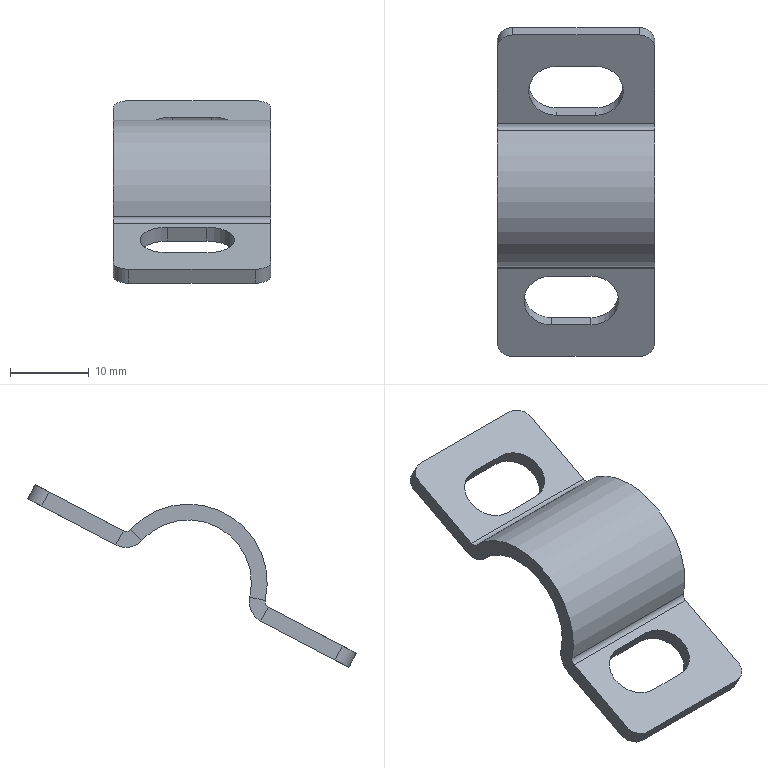Component | SolidWorks | SpringSnap-1 | 1 solid | 34 faces | box 20 x 41.66 x 23.15 mm | volume 1836 mm3 | plane 20 | cylinder 14 | commonest cylinder face diameters 7 x4 4 x4 5.473 x2 1.473 x2 16 x1 20 x1
STEP:
#1=COLOUR_RGB('',0.7922,0.8196,0.9333);
#2=FILL_AREA_STYLE_COLOUR('',#1);
#3=FILL_AREA_STYLE('',(#2));
#4=SURFACE_STYLE_FILL_AREA(#3);
#5=SURFACE_SIDE_STYLE('',(#4));
#6=SURFACE_STYLE_USAGE(.BOTH.,#5);
#7=PRESENTATION_STYLE_ASSIGNMENT((#6));
#8=CARTESIAN_POINT('',(-8.595,-0.65,7.005));
#9=VERTEX_POINT('',#8);
#10=CARTESIAN_POINT('',(-8.595,-0.592,7.058));
#11=VERTEX_POINT('',#10);
#12=CARTESIAN_POINT('',(-8.595,-0.65,7.005));
#13=DIRECTION('',(-0.,0.7377,0.6751));
#14=VECTOR('',#13,39.37);
#15=LINE('',#12,#14);
#16=EDGE_CURVE('',#9,#11,#15,.T.);
#17=ORIENTED_EDGE('',*,*,#16,.F.);
#18=CARTESIAN_POINT('',(-8.595,-0.5205,6.982));
#19=VERTEX_POINT('',#18);
#20=CARTESIAN_POINT('',(-8.595,-0.5706,7.078));
#21=DIRECTION('',(-1.,-0.,-0.));
#22=DIRECTION('',(0.,-0.8854,-0.4648));
#23=AXIS2_PLACEMENT_3D('',#20,#21,#22);
#24=CIRCLE('',#23,0.1077);
#25=EDGE_CURVE('',#19,#9,#24,.T.);
#26=ORIENTED_EDGE('',*,*,#25,.F.);
#27=CARTESIAN_POINT('',(-8.595,-0.5571,7.052));
#28=VERTEX_POINT('',#27);
#29=CARTESIAN_POINT('',(-8.595,-0.5571,7.052));
#30=DIRECTION('',(-0.,0.4648,-0.8854));
#31=VECTOR('',#30,39.37);
#32=LINE('',#29,#31);
#33=EDGE_CURVE('',#28,#19,#32,.T.);
#34=ORIENTED_EDGE('',*,*,#33,.F.);
#35=CARTESIAN_POINT('',(-8.595,-0.5706,7.078));
#36=DIRECTION('',(-1.,-0.,-0.));
#37=DIRECTION('',(0.,-0.8854,-0.4648));
#38=AXIS2_PLACEMENT_3D('',#35,#36,#37);
#39=CIRCLE('',#38,0.029);
#40=EDGE_CURVE('',#28,#11,#39,.T.);
#41=ORIENTED_EDGE('',*,*,#40,.T.);
#42=EDGE_LOOP('',(#17,#26,#34,#41));
#43=FACE_OUTER_BOUND('',#42,.T.);
#44=CARTESIAN_POINT('',(-8.595,-0.65,7.005));
#45=DIRECTION('',(1.,0.,0.));
#46=DIRECTION('',(0.,-0.8854,-0.4648));
#47=AXIS2_PLACEMENT_3D('',#44,#45,#46);
#48=PLANE('',#47);
#49=ADVANCED_FACE('',(#43),#48,.T.);
#50=CARTESIAN_POINT('',(-8.595,-1.189,6.722));
#51=VERTEX_POINT('',#50);
#52=CARTESIAN_POINT('',(-8.595,-0.8824,6.792));
#53=DIRECTION('',(1.,0.,0.));
#54=DIRECTION('',(0.,-0.8854,-0.4648));
#55=AXIS2_PLACEMENT_3D('',#52,#53,#54);
#56=CIRCLE('',#55,0.315);
#57=EDGE_CURVE('',#9,#51,#56,.T.);
#58=ORIENTED_EDGE('',*,*,#57,.F.);
#59=ORIENTED_EDGE('',*,*,#16,.T.);
#60=CARTESIAN_POINT('',(-8.595,-1.266,6.704));
#61=VERTEX_POINT('',#60);
#62=CARTESIAN_POINT('',(-8.595,-0.8824,6.792));
#63=DIRECTION('',(1.,0.,0.));
#64=DIRECTION('',(0.,-0.8854,-0.4648));
#65=AXIS2_PLACEMENT_3D('',#62,#63,#64);
#66=CIRCLE('',#65,0.3937);
#67=EDGE_CURVE('',#11,#61,#66,.T.);
#68=ORIENTED_EDGE('',*,*,#67,.T.);
#69=CARTESIAN_POINT('',(-8.595,-1.266,6.704));
#70=DIRECTION('',(-0.,0.9746,0.2238));
#71=VECTOR('',#70,39.37);
#72=LINE('',#69,#71);
#73=EDGE_CURVE('',#61,#51,#72,.T.);
#74=ORIENTED_EDGE('',*,*,#73,.T.);
#75=EDGE_LOOP('',(#58,#59,#68,#74));
#76=FACE_OUTER_BOUND('',#75,.T.);
#77=CARTESIAN_POINT('',(-8.595,-0.5571,7.052));
#78=DIRECTION('',(1.,0.,0.));
#79=DIRECTION('',(0.,-0.8854,-0.4648));
#80=AXIS2_PLACEMENT_3D('',#77,#78,#79);
#81=PLANE('',#80);
#82=ADVANCED_FACE('',(#76),#81,.T.);
#83=CARTESIAN_POINT('',(-9.383,-0.5205,6.982));
#84=VERTEX_POINT('',#83);
#85=CARTESIAN_POINT('',(-9.383,-0.5571,7.052));
#86=VERTEX_POINT('',#85);
#87=CARTESIAN_POINT('',(-9.383,-0.5205,6.982));
#88=DIRECTION('',(0.,-0.4648,0.8854));
#89=VECTOR('',#88,39.37);
#90=LINE('',#87,#89);
#91=EDGE_CURVE('',#84,#86,#90,.T.);
#92=ORIENTED_EDGE('',*,*,#91,.F.);
#93=CARTESIAN_POINT('',(-9.383,-0.65,7.005));
#94=VERTEX_POINT('',#93);
#95=CARTESIAN_POINT('',(-9.383,-0.5706,7.078));
#96=DIRECTION('',(-1.,-0.,-0.));
#97=DIRECTION('',(0.,-0.8854,-0.4648));
#98=AXIS2_PLACEMENT_3D('',#95,#96,#97);
#99=CIRCLE('',#98,0.1077);
#100=EDGE_CURVE('',#84,#94,#99,.T.);
#101=ORIENTED_EDGE('',*,*,#100,.T.);
#102=CARTESIAN_POINT('',(-9.383,-0.592,7.058));
#103=VERTEX_POINT('',#102);
#104=CARTESIAN_POINT('',(-9.383,-0.592,7.058));
#105=DIRECTION('',(0.,-0.7377,-0.6751));
#106=VECTOR('',#105,39.37);
#107=LINE('',#104,#106);
#108=EDGE_CURVE('',#103,#94,#107,.T.);
#109=ORIENTED_EDGE('',*,*,#108,.F.);
#110=CARTESIAN_POINT('',(-9.383,-0.5706,7.078));
#111=DIRECTION('',(-1.,-0.,-0.));
#112=DIRECTION('',(0.,-0.8854,-0.4648));
#113=AXIS2_PLACEMENT_3D('',#110,#111,#112);
#114=CIRCLE('',#113,0.029);
#115=EDGE_CURVE('',#86,#103,#114,.T.);
#116=ORIENTED_EDGE('',*,*,#115,.F.);
#117=EDGE_LOOP('',(#92,#101,#109,#116));
#118=FACE_OUTER_BOUND('',#117,.T.);
#119=CARTESIAN_POINT('',(-9.383,-0.5205,6.982));
#120=DIRECTION('',(-1.,-0.,-0.));
#121=DIRECTION('',(-0.,0.8854,0.4648));
#122=AXIS2_PLACEMENT_3D('',#119,#120,#121);
#123=PLANE('',#122);
#124=ADVANCED_FACE('',(#118),#123,.T.);
#125=CARTESIAN_POINT('',(-9.383,-0.187,7.246));
#126=VERTEX_POINT('',#125);
#127=CARTESIAN_POINT('',(-9.383,-0.6401,7.008));
#128=DIRECTION('',(0.,-0.8854,-0.4648));
#129=VECTOR('',#128,39.37);
#130=LINE('',#127,#129);
#131=EDGE_CURVE('',#126,#86,#130,.T.);
#132=ORIENTED_EDGE('',*,*,#131,.F.);
#133=CARTESIAN_POINT('',(-9.383,-0.1504,7.177));
#134=VERTEX_POINT('',#133);
#135=CARTESIAN_POINT('',(-9.383,-0.197,7.265));
#136=DIRECTION('',(-0.,0.4648,-0.8854));
#137=VECTOR('',#136,39.37);
#138=LINE('',#135,#137);
#139=EDGE_CURVE('',#126,#134,#138,.T.);
#140=ORIENTED_EDGE('',*,*,#139,.T.);
#141=CARTESIAN_POINT('',(-9.383,-0.6035,6.939));
#142=DIRECTION('',(0.,-0.8854,-0.4648));
#143=VECTOR('',#142,39.37);
#144=LINE('',#141,#143);
#145=EDGE_CURVE('',#134,#84,#144,.T.);
#146=ORIENTED_EDGE('',*,*,#145,.T.);
#147=ORIENTED_EDGE('',*,*,#91,.T.);
#148=EDGE_LOOP('',(#132,#140,#146,#147));
#149=FACE_OUTER_BOUND('',#148,.T.);
#150=CARTESIAN_POINT('',(-9.383,-0.592,7.058));
#151=DIRECTION('',(-1.,-0.,-0.));
#152=DIRECTION('',(-0.,0.8854,0.4648));
#153=AXIS2_PLACEMENT_3D('',#150,#151,#152);
#154=PLANE('',#153);
#155=ADVANCED_FACE('',(#149),#154,.T.);
#156=CARTESIAN_POINT('',(-8.595,-1.244,6.602));
#157=VERTEX_POINT('',#156);
#158=CARTESIAN_POINT('',(-8.595,-1.281,6.672));
#159=VERTEX_POINT('',#158);
#160=CARTESIAN_POINT('',(-8.595,-1.244,6.602));
#161=DIRECTION('',(0.,-0.4648,0.8854));
#162=VECTOR('',#161,39.37);
#163=LINE('',#160,#162);
#164=EDGE_CURVE('',#157,#159,#163,.T.);
#165=ORIENTED_EDGE('',*,*,#164,.F.);
#166=CARTESIAN_POINT('',(-8.595,-1.294,6.698));
#167=DIRECTION('',(-1.,-0.,-0.));
#168=DIRECTION('',(0.,-0.8854,-0.4648));
#169=AXIS2_PLACEMENT_3D('',#166,#167,#168);
#170=CIRCLE('',#169,0.1077);
#171=EDGE_CURVE('',#51,#157,#170,.T.);
#172=ORIENTED_EDGE('',*,*,#171,.F.);
#173=ORIENTED_EDGE('',*,*,#73,.F.);
#174=CARTESIAN_POINT('',(-8.595,-1.294,6.698));
#175=DIRECTION('',(-1.,-0.,-0.));
#176=DIRECTION('',(0.,-0.8854,-0.4648));
#177=AXIS2_PLACEMENT_3D('',#174,#175,#176);
#178=CIRCLE('',#177,0.029);
#179=EDGE_CURVE('',#61,#159,#178,.T.);
#180=ORIENTED_EDGE('',*,*,#179,.T.);
#181=EDGE_LOOP('',(#165,#172,#173,#180));
#182=FACE_OUTER_BOUND('',#181,.T.);
#183=CARTESIAN_POINT('',(-8.595,-1.244,6.602));
#184=DIRECTION('',(1.,0.,0.));
#185=DIRECTION('',(0.,-0.8854,-0.4648));
#186=AXIS2_PLACEMENT_3D('',#183,#184,#185);
#187=PLANE('',#186);
#188=ADVANCED_FACE('',(#182),#187,.T.);
#189=CARTESIAN_POINT('',(-8.595,-1.651,6.478));
#190=VERTEX_POINT('',#189);
#191=CARTESIAN_POINT('',(-8.595,-1.198,6.716));
#192=DIRECTION('',(0.,-0.8854,-0.4648));
#193=VECTOR('',#192,39.37);
#194=LINE('',#191,#193);
#195=EDGE_CURVE('',#159,#190,#194,.T.);
#196=ORIENTED_EDGE('',*,*,#195,.T.);
#197=CARTESIAN_POINT('',(-8.595,-1.614,6.408));
#198=VERTEX_POINT('',#197);
#199=CARTESIAN_POINT('',(-8.595,-1.661,6.497));
#200=DIRECTION('',(-0.,0.4648,-0.8854));
#201=VECTOR('',#200,39.37);
#202=LINE('',#199,#201);
#203=EDGE_CURVE('',#190,#198,#202,.T.);
#204=ORIENTED_EDGE('',*,*,#203,.T.);
#205=CARTESIAN_POINT('',(-8.595,-1.161,6.646));
#206=DIRECTION('',(0.,-0.8854,-0.4648));
#207=VECTOR('',#206,39.37);
#208=LINE('',#205,#207);
#209=EDGE_CURVE('',#157,#198,#208,.T.);
#210=ORIENTED_EDGE('',*,*,#209,.F.);
#211=ORIENTED_EDGE('',*,*,#164,.T.);
#212=EDGE_LOOP('',(#196,#204,#210,#211));
#213=FACE_OUTER_BOUND('',#212,.T.);
#214=CARTESIAN_POINT('',(-8.595,-1.266,6.704));
#215=DIRECTION('',(1.,0.,0.));
#216=DIRECTION('',(0.,-0.8854,-0.4648));
#217=AXIS2_PLACEMENT_3D('',#214,#215,#216);
#218=PLANE('',#217);
#219=ADVANCED_FACE('',(#213),#218,.T.);
#220=CARTESIAN_POINT('',(-9.383,-1.189,6.722));
#221=VERTEX_POINT('',#220);
#222=CARTESIAN_POINT('',(-9.383,-1.266,6.704));
#223=VERTEX_POINT('',#222);
#224=CARTESIAN_POINT('',(-9.383,-1.189,6.722));
#225=DIRECTION('',(0.,-0.9746,-0.2238));
#226=VECTOR('',#225,39.37);
#227=LINE('',#224,#226);
#228=EDGE_CURVE('',#221,#223,#227,.T.);
#229=ORIENTED_EDGE('',*,*,#228,.F.);
#230=CARTESIAN_POINT('',(-9.383,-1.244,6.602));
#231=VERTEX_POINT('',#230);
#232=CARTESIAN_POINT('',(-9.383,-1.294,6.698));
#233=DIRECTION('',(-1.,-0.,-0.));
#234=DIRECTION('',(0.,-0.8854,-0.4648));
#235=AXIS2_PLACEMENT_3D('',#232,#233,#234);
#236=CIRCLE('',#235,0.1077);
#237=EDGE_CURVE('',#221,#231,#236,.T.);
#238=ORIENTED_EDGE('',*,*,#237,.T.);
#239=CARTESIAN_POINT('',(-9.383,-1.281,6.672));
#240=VERTEX_POINT('',#239);
#241=CARTESIAN_POINT('',(-9.383,-1.281,6.672));
#242=DIRECTION('',(-0.,0.4648,-0.8854));
#243=VECTOR('',#242,39.37);
#244=LINE('',#241,#243);
#245=EDGE_CURVE('',#240,#231,#244,.T.);
#246=ORIENTED_EDGE('',*,*,#245,.F.);
#247=CARTESIAN_POINT('',(-9.383,-1.294,6.698));
#248=DIRECTION('',(-1.,-0.,-0.));
#249=DIRECTION('',(0.,-0.8854,-0.4648));
#250=AXIS2_PLACEMENT_3D('',#247,#248,#249);
#251=CIRCLE('',#250,0.029);
#252=EDGE_CURVE('',#223,#240,#251,.T.);
#253=ORIENTED_EDGE('',*,*,#252,.F.);
#254=EDGE_LOOP('',(#229,#238,#246,#253));
#255=FACE_OUTER_BOUND('',#254,.T.);
#256=CARTESIAN_POINT('',(-9.383,-1.189,6.722));
#257=DIRECTION('',(-1.,-0.,-0.));
#258=DIRECTION('',(-0.,0.8854,0.4648));
#259=AXIS2_PLACEMENT_3D('',#256,#257,#258);
#260=PLANE('',#259);
#261=ADVANCED_FACE('',(#255),#260,.T.);
#262=CARTESIAN_POINT('',(-9.383,-0.8824,6.792));
#263=DIRECTION('',(1.,0.,0.));
#264=DIRECTION('',(0.,-0.8854,-0.4648));
#265=AXIS2_PLACEMENT_3D('',#262,#263,#264);
#266=CIRCLE('',#265,0.315);
#267=EDGE_CURVE('',#94,#221,#266,.T.);
#268=ORIENTED_EDGE('',*,*,#267,.T.);
#269=ORIENTED_EDGE('',*,*,#228,.T.);
#270=CARTESIAN_POINT('',(-9.383,-0.8824,6.792));
#271=DIRECTION('',(1.,0.,0.));
#272=DIRECTION('',(0.,-0.8854,-0.4648));
#273=AXIS2_PLACEMENT_3D('',#270,#271,#272);
#274=CIRCLE('',#273,0.3937);
#275=EDGE_CURVE('',#103,#223,#274,.T.);
#276=ORIENTED_EDGE('',*,*,#275,.F.);
#277=ORIENTED_EDGE('',*,*,#108,.T.);
#278=EDGE_LOOP('',(#268,#269,#276,#277));
#279=FACE_OUTER_BOUND('',#278,.T.);
#280=CARTESIAN_POINT('',(-9.383,-1.281,6.672));
#281=DIRECTION('',(-1.,-0.,-0.));
#282=DIRECTION('',(-0.,0.8854,0.4648));
#283=AXIS2_PLACEMENT_3D('',#280,#281,#282);
#284=PLANE('',#283);
#285=ADVANCED_FACE('',(#279),#284,.T.);
#286=CARTESIAN_POINT('',(-8.914,-1.32,6.652));
#287=VERTEX_POINT('',#286);
#288=CARTESIAN_POINT('',(-9.111,-1.32,6.652));
#289=VERTEX_POINT('',#288);
#290=CARTESIAN_POINT('',(-8.914,-1.32,6.652));
#291=DIRECTION('',(-1.,-0.,-0.));
#292=VECTOR('',#291,39.37);
#293=LINE('',#290,#292);
#294=EDGE_CURVE('',#287,#289,#293,.T.);
#295=ORIENTED_EDGE('',*,*,#294,.F.);
#296=CARTESIAN_POINT('',(-8.914,-1.564,6.523));
#297=VERTEX_POINT('',#296);
#298=CARTESIAN_POINT('',(-8.914,-1.442,6.587));
#299=DIRECTION('',(0.,-0.4648,0.8854));
#300=DIRECTION('',(0.,-0.8854,-0.4648));
#301=AXIS2_PLACEMENT_3D('',#298,#299,#300);
#302=CIRCLE('',#301,0.1378);
#303=EDGE_CURVE('',#297,#287,#302,.T.);
#304=ORIENTED_EDGE('',*,*,#303,.F.);
#305=CARTESIAN_POINT('',(-9.111,-1.564,6.523));
#306=VERTEX_POINT('',#305);
#307=CARTESIAN_POINT('',(-8.914,-1.564,6.523));
#308=DIRECTION('',(1.,0.,0.));
#309=VECTOR('',#308,39.37);
#310=LINE('',#307,#309);
#311=EDGE_CURVE('',#306,#297,#310,.T.);
#312=ORIENTED_EDGE('',*,*,#311,.F.);
#313=CARTESIAN_POINT('',(-9.111,-1.442,6.587));
#314=DIRECTION('',(0.,-0.4648,0.8854));
#315=DIRECTION('',(0.,-0.8854,-0.4648));
#316=AXIS2_PLACEMENT_3D('',#313,#314,#315);
#317=CIRCLE('',#316,0.1378);
#318=EDGE_CURVE('',#289,#306,#317,.T.);
#319=ORIENTED_EDGE('',*,*,#318,.F.);
#320=EDGE_LOOP('',(#295,#304,#312,#319));
#321=FACE_BOUND('',#320,.T.);
#322=CARTESIAN_POINT('',(-8.674,-1.721,6.441));
#323=VERTEX_POINT('',#322);
#324=CARTESIAN_POINT('',(-9.304,-1.721,6.441));
#325=VERTEX_POINT('',#324);
#326=CARTESIAN_POINT('',(-8.595,-1.721,6.441));
#327=DIRECTION('',(-1.,-0.,-0.));
#328=VECTOR('',#327,39.37);
#329=LINE('',#326,#328);
#330=EDGE_CURVE('',#323,#325,#329,.T.);
#331=ORIENTED_EDGE('',*,*,#330,.F.);
#332=CARTESIAN_POINT('',(-8.674,-1.651,6.478));
#333=DIRECTION('',(0.,-0.4648,0.8854));
#334=DIRECTION('',(1.,0.,0.));
#335=AXIS2_PLACEMENT_3D('',#332,#333,#334);
#336=CIRCLE('',#335,0.07874);
#337=EDGE_CURVE('',#323,#190,#336,.T.);
#338=ORIENTED_EDGE('',*,*,#337,.T.);
#339=ORIENTED_EDGE('',*,*,#195,.F.);
#340=CARTESIAN_POINT('',(-8.595,-1.281,6.672));
#341=DIRECTION('',(-1.,-0.,-0.));
#342=VECTOR('',#341,39.37);
#343=LINE('',#340,#342);
#344=EDGE_CURVE('',#159,#240,#343,.T.);
#345=ORIENTED_EDGE('',*,*,#344,.T.);
#346=CARTESIAN_POINT('',(-9.383,-1.651,6.478));
#347=VERTEX_POINT('',#346);
#348=CARTESIAN_POINT('',(-9.383,-1.198,6.716));
#349=DIRECTION('',(0.,-0.8854,-0.4648));
#350=VECTOR('',#349,39.37);
#351=LINE('',#348,#350);
#352=EDGE_CURVE('',#240,#347,#351,.T.);
#353=ORIENTED_EDGE('',*,*,#352,.T.);
#354=CARTESIAN_POINT('',(-9.304,-1.651,6.478));
#355=DIRECTION('',(0.,-0.4648,0.8854));
#356=DIRECTION('',(1.,0.,0.));
#357=AXIS2_PLACEMENT_3D('',#354,#355,#356);
#358=CIRCLE('',#357,0.07874);
#359=EDGE_CURVE('',#347,#325,#358,.T.);
#360=ORIENTED_EDGE('',*,*,#359,.T.);
#361=EDGE_LOOP('',(#331,#338,#339,#345,#353,#360));
#362=FACE_OUTER_BOUND('',#361,.T.);
#363=CARTESIAN_POINT('',(-8.595,-1.198,6.716));
#364=DIRECTION('',(-0.,0.4648,-0.8854));
#365=DIRECTION('',(1.,0.,0.));
#366=AXIS2_PLACEMENT_3D('',#363,#364,#365);
#367=PLANE('',#366);
#368=ADVANCED_FACE('',(#321,#362),#367,.F.);
#369=CARTESIAN_POINT('',(-8.674,-1.684,6.371));
#370=VERTEX_POINT('',#369);
#371=CARTESIAN_POINT('',(-9.304,-1.684,6.371));
#372=VERTEX_POINT('',#371);
#373=CARTESIAN_POINT('',(-8.595,-1.684,6.371));
#374=DIRECTION('',(-1.,-0.,-0.));
#375=VECTOR('',#374,39.37);
#376=LINE('',#373,#375);
#377=EDGE_CURVE('',#370,#372,#376,.T.);
#378=ORIENTED_EDGE('',*,*,#377,.F.);
#379=CARTESIAN_POINT('',(-8.674,-1.684,6.371));
#380=DIRECTION('',(0.,-0.4648,0.8854));
#381=VECTOR('',#380,39.37);
#382=LINE('',#379,#381);
#383=EDGE_CURVE('',#370,#323,#382,.T.);
#384=ORIENTED_EDGE('',*,*,#383,.T.);
#385=ORIENTED_EDGE('',*,*,#330,.T.);
#386=CARTESIAN_POINT('',(-9.304,-1.684,6.371));
#387=DIRECTION('',(-0.,0.4648,-0.8854));
#388=VECTOR('',#387,39.37);
#389=LINE('',#386,#388);
#390=EDGE_CURVE('',#325,#372,#389,.T.);
#391=ORIENTED_EDGE('',*,*,#390,.T.);
#392=EDGE_LOOP('',(#378,#384,#385,#391));
#393=FACE_OUTER_BOUND('',#392,.T.);
#394=CARTESIAN_POINT('',(-8.595,-1.684,6.371));
#395=DIRECTION('',(0.,-0.8854,-0.4648));
#396=DIRECTION('',(-1.,-0.,-0.));
#397=AXIS2_PLACEMENT_3D('',#394,#395,#396);
#398=PLANE('',#397);
#399=ADVANCED_FACE('',(#393),#398,.T.);
#400=CARTESIAN_POINT('',(-8.914,-1.283,6.582));
#401=VERTEX_POINT('',#400);
#402=CARTESIAN_POINT('',(-8.914,-1.527,6.454));
#403=VERTEX_POINT('',#402);
#404=CARTESIAN_POINT('',(-8.914,-1.405,6.518));
#405=DIRECTION('',(-0.,0.4648,-0.8854));
#406=DIRECTION('',(1.,0.,0.));
#407=AXIS2_PLACEMENT_3D('',#404,#405,#406);
#408=CIRCLE('',#407,0.1378);
#409=EDGE_CURVE('',#401,#403,#408,.T.);
#410=ORIENTED_EDGE('',*,*,#409,.F.);
#411=CARTESIAN_POINT('',(-9.111,-1.283,6.582));
#412=VERTEX_POINT('',#411);
#413=CARTESIAN_POINT('',(-8.595,-1.283,6.582));
#414=DIRECTION('',(1.,0.,0.));
#415=VECTOR('',#414,39.37);
#416=LINE('',#413,#415);
#417=EDGE_CURVE('',#412,#401,#416,.T.);
#418=ORIENTED_EDGE('',*,*,#417,.F.);
#419=CARTESIAN_POINT('',(-9.111,-1.527,6.454));
#420=VERTEX_POINT('',#419);
#421=CARTESIAN_POINT('',(-9.111,-1.405,6.518));
#422=DIRECTION('',(-0.,0.4648,-0.8854));
#423=DIRECTION('',(1.,0.,0.));
#424=AXIS2_PLACEMENT_3D('',#421,#422,#423);
#425=CIRCLE('',#424,0.1378);
#426=EDGE_CURVE('',#420,#412,#425,.T.);
#427=ORIENTED_EDGE('',*,*,#426,.F.);
#428=CARTESIAN_POINT('',(-8.595,-1.527,6.454));
#429=DIRECTION('',(-1.,-0.,-0.));
#430=VECTOR('',#429,39.37);
#431=LINE('',#428,#430);
#432=EDGE_CURVE('',#403,#420,#431,.T.);
#433=ORIENTED_EDGE('',*,*,#432,.F.);
#434=EDGE_LOOP('',(#410,#418,#427,#433));
#435=FACE_BOUND('',#434,.T.);
#436=ORIENTED_EDGE('',*,*,#209,.T.);
#437=CARTESIAN_POINT('',(-8.674,-1.614,6.408));
#438=DIRECTION('',(-0.,0.4648,-0.8854));
#439=DIRECTION('',(1.,0.,0.));
#440=AXIS2_PLACEMENT_3D('',#437,#438,#439);
#441=CIRCLE('',#440,0.07874);
#442=EDGE_CURVE('',#198,#370,#441,.T.);
#443=ORIENTED_EDGE('',*,*,#442,.T.);
#444=ORIENTED_EDGE('',*,*,#377,.T.);
#445=CARTESIAN_POINT('',(-9.383,-1.614,6.408));
#446=VERTEX_POINT('',#445);
#447=CARTESIAN_POINT('',(-9.304,-1.614,6.408));
#448=DIRECTION('',(-0.,0.4648,-0.8854));
#449=DIRECTION('',(1.,0.,0.));
#450=AXIS2_PLACEMENT_3D('',#447,#448,#449);
#451=CIRCLE('',#450,0.07874);
#452=EDGE_CURVE('',#372,#446,#451,.T.);
#453=ORIENTED_EDGE('',*,*,#452,.T.);
#454=CARTESIAN_POINT('',(-9.383,-1.161,6.646));
#455=DIRECTION('',(0.,-0.8854,-0.4648));
#456=VECTOR('',#455,39.37);
#457=LINE('',#454,#456);
#458=EDGE_CURVE('',#231,#446,#457,.T.);
#459=ORIENTED_EDGE('',*,*,#458,.F.);
#460=CARTESIAN_POINT('',(-8.595,-1.244,6.602));
#461=DIRECTION('',(-1.,-0.,-0.));
#462=VECTOR('',#461,39.37);
#463=LINE('',#460,#462);
#464=EDGE_CURVE('',#157,#231,#463,.T.);
#465=ORIENTED_EDGE('',*,*,#464,.F.);
#466=EDGE_LOOP('',(#436,#443,#444,#453,#459,#465));
#467=FACE_OUTER_BOUND('',#466,.T.);
#468=CARTESIAN_POINT('',(-8.595,-1.161,6.646));
#469=DIRECTION('',(-0.,0.4648,-0.8854));
#470=DIRECTION('',(1.,0.,0.));
#471=AXIS2_PLACEMENT_3D('',#468,#469,#470);
#472=PLANE('',#471);
#473=ADVANCED_FACE('',(#435,#467),#472,.T.);
#474=ORIENTED_EDGE('',*,*,#237,.F.);
#475=CARTESIAN_POINT('',(-8.595,-1.189,6.722));
#476=DIRECTION('',(-1.,-0.,-0.));
#477=VECTOR('',#476,39.37);
#478=LINE('',#475,#477);
#479=EDGE_CURVE('',#51,#221,#478,.T.);
#480=ORIENTED_EDGE('',*,*,#479,.F.);
#481=ORIENTED_EDGE('',*,*,#171,.T.);
#482=ORIENTED_EDGE('',*,*,#464,.T.);
#483=EDGE_LOOP('',(#474,#480,#481,#482));
#484=FACE_OUTER_BOUND('',#483,.T.);
#485=CARTESIAN_POINT('',(-8.595,-1.294,6.698));
#486=DIRECTION('',(-1.,-0.,-0.));
#487=DIRECTION('',(0.,0.8854,0.4648));
#488=AXIS2_PLACEMENT_3D('',#485,#486,#487);
#489=CYLINDRICAL_SURFACE('',#488,0.1077);
#490=ADVANCED_FACE('',(#484),#489,.T.);
#491=ORIENTED_EDGE('',*,*,#267,.F.);
#492=CARTESIAN_POINT('',(-8.595,-0.65,7.005));
#493=DIRECTION('',(-1.,-0.,-0.));
#494=VECTOR('',#493,39.37);
#495=LINE('',#492,#494);
#496=EDGE_CURVE('',#9,#94,#495,.T.);
#497=ORIENTED_EDGE('',*,*,#496,.F.);
#498=ORIENTED_EDGE('',*,*,#57,.T.);
#499=ORIENTED_EDGE('',*,*,#479,.T.);
#500=EDGE_LOOP('',(#491,#497,#498,#499));
#501=FACE_OUTER_BOUND('',#500,.T.);
#502=CARTESIAN_POINT('',(-8.595,-0.8824,6.792));
#503=DIRECTION('',(-1.,-0.,-0.));
#504=DIRECTION('',(-0.,0.8854,0.4648));
#505=AXIS2_PLACEMENT_3D('',#502,#503,#504);
#506=CYLINDRICAL_SURFACE('',#505,0.315);
#507=ADVANCED_FACE('',(#501),#506,.F.);
#508=ORIENTED_EDGE('',*,*,#100,.F.);
#509=CARTESIAN_POINT('',(-8.595,-0.5205,6.982));
#510=DIRECTION('',(-1.,-0.,-0.));
#511=VECTOR('',#510,39.37);
#512=LINE('',#509,#511);
#513=EDGE_CURVE('',#19,#84,#512,.T.);
#514=ORIENTED_EDGE('',*,*,#513,.F.);
#515=ORIENTED_EDGE('',*,*,#25,.T.);
#516=ORIENTED_EDGE('',*,*,#496,.T.);
#517=EDGE_LOOP('',(#508,#514,#515,#516));
#518=FACE_OUTER_BOUND('',#517,.T.);
#519=CARTESIAN_POINT('',(-8.595,-0.5706,7.078));
#520=DIRECTION('',(-1.,-0.,-0.));
#521=DIRECTION('',(0.,0.8854,0.4648));
#522=AXIS2_PLACEMENT_3D('',#519,#520,#521);
#523=CYLINDRICAL_SURFACE('',#522,0.1077);
#524=ADVANCED_FACE('',(#518),#523,.T.);
#525=CARTESIAN_POINT('',(-8.891,-0.2375,7.131));
#526=VERTEX_POINT('',#525);
#527=CARTESIAN_POINT('',(-8.891,-0.4815,7.003));
#528=VERTEX_POINT('',#527);
#529=CARTESIAN_POINT('',(-8.891,-0.3595,7.067));
#530=DIRECTION('',(-0.,0.4648,-0.8854));
#531=DIRECTION('',(0.,0.8854,0.4648));
#532=AXIS2_PLACEMENT_3D('',#529,#530,#531);
#533=CIRCLE('',#532,0.1378);
#534=EDGE_CURVE('',#526,#528,#533,.T.);
#535=ORIENTED_EDGE('',*,*,#534,.F.);
#536=CARTESIAN_POINT('',(-9.087,-0.2375,7.131));
#537=VERTEX_POINT('',#536);
#538=CARTESIAN_POINT('',(-8.595,-0.2375,7.131));
#539=DIRECTION('',(1.,0.,0.));
#540=VECTOR('',#539,39.37);
#541=LINE('',#538,#540);
#542=EDGE_CURVE('',#537,#526,#541,.T.);
#543=ORIENTED_EDGE('',*,*,#542,.F.);
#544=CARTESIAN_POINT('',(-9.087,-0.4815,7.003));
#545=VERTEX_POINT('',#544);
#546=CARTESIAN_POINT('',(-9.087,-0.3595,7.067));
#547=DIRECTION('',(-0.,0.4648,-0.8854));
#548=DIRECTION('',(0.,0.8854,0.4648));
#549=AXIS2_PLACEMENT_3D('',#546,#547,#548);
#550=CIRCLE('',#549,0.1378);
#551=EDGE_CURVE('',#545,#537,#550,.T.);
#552=ORIENTED_EDGE('',*,*,#551,.F.);
#553=CARTESIAN_POINT('',(-8.595,-0.4815,7.003));
#554=DIRECTION('',(-1.,-0.,-0.));
#555=VECTOR('',#554,39.37);
#556=LINE('',#553,#555);
#557=EDGE_CURVE('',#528,#545,#556,.T.);
#558=ORIENTED_EDGE('',*,*,#557,.F.);
#559=EDGE_LOOP('',(#535,#543,#552,#558));
#560=FACE_BOUND('',#559,.T.);
#561=CARTESIAN_POINT('',(-8.674,-0.08064,7.213));
#562=VERTEX_POINT('',#561);
#563=CARTESIAN_POINT('',(-9.304,-0.08064,7.213));
#564=VERTEX_POINT('',#563);
#565=CARTESIAN_POINT('',(-8.595,-0.08064,7.213));
#566=DIRECTION('',(-1.,-0.,-0.));
#567=VECTOR('',#566,39.37);
#568=LINE('',#565,#567);
#569=EDGE_CURVE('',#562,#564,#568,.T.);
#570=ORIENTED_EDGE('',*,*,#569,.F.);
#571=CARTESIAN_POINT('',(-8.595,-0.1504,7.177));
#572=VERTEX_POINT('',#571);
#573=CARTESIAN_POINT('',(-8.674,-0.1504,7.177));
#574=DIRECTION('',(-0.,0.4648,-0.8854));
#575=DIRECTION('',(0.,0.8854,0.4648));
#576=AXIS2_PLACEMENT_3D('',#573,#574,#575);
#577=CIRCLE('',#576,0.07874);
#578=EDGE_CURVE('',#562,#572,#577,.T.);
#579=ORIENTED_EDGE('',*,*,#578,.T.);
#580=CARTESIAN_POINT('',(-8.595,-0.6035,6.939));
#581=DIRECTION('',(0.,-0.8854,-0.4648));
#582=VECTOR('',#581,39.37);
#583=LINE('',#580,#582);
#584=EDGE_CURVE('',#572,#19,#583,.T.);
#585=ORIENTED_EDGE('',*,*,#584,.T.);
#586=ORIENTED_EDGE('',*,*,#513,.T.);
#587=ORIENTED_EDGE('',*,*,#145,.F.);
#588=CARTESIAN_POINT('',(-9.304,-0.1504,7.177));
#589=DIRECTION('',(-0.,0.4648,-0.8854));
#590=DIRECTION('',(0.,0.8854,0.4648));
#591=AXIS2_PLACEMENT_3D('',#588,#589,#590);
#592=CIRCLE('',#591,0.07874);
#593=EDGE_CURVE('',#134,#564,#592,.T.);
#594=ORIENTED_EDGE('',*,*,#593,.T.);
#595=EDGE_LOOP('',(#570,#579,#585,#586,#587,#594));
#596=FACE_OUTER_BOUND('',#595,.T.);
#597=CARTESIAN_POINT('',(-8.595,-0.6035,6.939));
#598=DIRECTION('',(-0.,0.4648,-0.8854));
#599=DIRECTION('',(-0.,0.8854,0.4648));
#600=AXIS2_PLACEMENT_3D('',#597,#598,#599);
#601=PLANE('',#600);
#602=ADVANCED_FACE('',(#560,#596),#601,.T.);
#603=CARTESIAN_POINT('',(-8.674,-0.1172,7.283));
#604=VERTEX_POINT('',#603);
#605=CARTESIAN_POINT('',(-9.304,-0.1172,7.283));
#606=VERTEX_POINT('',#605);
#607=CARTESIAN_POINT('',(-8.595,-0.1172,7.283));
#608=DIRECTION('',(-1.,-0.,-0.));
#609=VECTOR('',#608,39.37);
#610=LINE('',#607,#609);
#611=EDGE_CURVE('',#604,#606,#610,.T.);
#612=ORIENTED_EDGE('',*,*,#611,.F.);
#613=CARTESIAN_POINT('',(-8.674,-0.1172,7.283));
#614=DIRECTION('',(-0.,0.4648,-0.8854));
#615=VECTOR('',#614,39.37);
#616=LINE('',#613,#615);
#617=EDGE_CURVE('',#604,#562,#616,.T.);
#618=ORIENTED_EDGE('',*,*,#617,.T.);
#619=ORIENTED_EDGE('',*,*,#569,.T.);
#620=CARTESIAN_POINT('',(-9.304,-0.1172,7.283));
#621=DIRECTION('',(0.,-0.4648,0.8854));
#622=VECTOR('',#621,39.37);
#623=LINE('',#620,#622);
#624=EDGE_CURVE('',#564,#606,#623,.T.);
#625=ORIENTED_EDGE('',*,*,#624,.T.);
#626=EDGE_LOOP('',(#612,#618,#619,#625));
#627=FACE_OUTER_BOUND('',#626,.T.);
#628=CARTESIAN_POINT('',(-8.595,-0.1172,7.283));
#629=DIRECTION('',(-0.,0.8854,0.4648));
#630=DIRECTION('',(1.,0.,0.));
#631=AXIS2_PLACEMENT_3D('',#628,#629,#630);
#632=PLANE('',#631);
#633=ADVANCED_FACE('',(#627),#632,.T.);
#634=CARTESIAN_POINT('',(-8.891,-0.2741,7.201));
#635=VERTEX_POINT('',#634);
#636=CARTESIAN_POINT('',(-9.087,-0.2741,7.201));
#637=VERTEX_POINT('',#636);
#638=CARTESIAN_POINT('',(-8.891,-0.2741,7.201));
#639=DIRECTION('',(-1.,-0.,-0.));
#640=VECTOR('',#639,39.37);
#641=LINE('',#638,#640);
#642=EDGE_CURVE('',#635,#637,#641,.T.);
#643=ORIENTED_EDGE('',*,*,#642,.F.);
#644=CARTESIAN_POINT('',(-8.891,-0.5181,7.072));
#645=VERTEX_POINT('',#644);
#646=CARTESIAN_POINT('',(-8.891,-0.3961,7.136));
#647=DIRECTION('',(0.,-0.4648,0.8854));
#648=DIRECTION('',(0.,-0.8854,-0.4648));
#649=AXIS2_PLACEMENT_3D('',#646,#647,#648);
#650=CIRCLE('',#649,0.1378);
#651=EDGE_CURVE('',#645,#635,#650,.T.);
#652=ORIENTED_EDGE('',*,*,#651,.F.);
#653=CARTESIAN_POINT('',(-9.087,-0.5181,7.072));
#654=VERTEX_POINT('',#653);
#655=CARTESIAN_POINT('',(-8.891,-0.5181,7.072));
#656=DIRECTION('',(1.,0.,0.));
#657=VECTOR('',#656,39.37);
#658=LINE('',#655,#657);
#659=EDGE_CURVE('',#654,#645,#658,.T.);
#660=ORIENTED_EDGE('',*,*,#659,.F.);
#661=CARTESIAN_POINT('',(-9.087,-0.3961,7.136));
#662=DIRECTION('',(0.,-0.4648,0.8854));
#663=DIRECTION('',(0.,-0.8854,-0.4648));
#664=AXIS2_PLACEMENT_3D('',#661,#662,#663);
#665=CIRCLE('',#664,0.1378);
#666=EDGE_CURVE('',#637,#654,#665,.T.);
#667=ORIENTED_EDGE('',*,*,#666,.F.);
#668=EDGE_LOOP('',(#643,#652,#660,#667));
#669=FACE_BOUND('',#668,.T.);
#670=CARTESIAN_POINT('',(-8.595,-0.187,7.246));
#671=VERTEX_POINT('',#670);
#672=CARTESIAN_POINT('',(-8.595,-0.6401,7.008));
#673=DIRECTION('',(0.,-0.8854,-0.4648));
#674=VECTOR('',#673,39.37);
#675=LINE('',#672,#674);
#676=EDGE_CURVE('',#671,#28,#675,.T.);
#677=ORIENTED_EDGE('',*,*,#676,.F.);
#678=CARTESIAN_POINT('',(-8.674,-0.187,7.246));
#679=DIRECTION('',(0.,-0.4648,0.8854));
#680=DIRECTION('',(0.,0.8854,0.4648));
#681=AXIS2_PLACEMENT_3D('',#678,#679,#680);
#682=CIRCLE('',#681,0.07874);
#683=EDGE_CURVE('',#671,#604,#682,.T.);
#684=ORIENTED_EDGE('',*,*,#683,.T.);
#685=ORIENTED_EDGE('',*,*,#611,.T.);
#686=CARTESIAN_POINT('',(-9.304,-0.187,7.246));
#687=DIRECTION('',(0.,-0.4648,0.8854));
#688=DIRECTION('',(-0.,0.8854,0.4648));
#689=AXIS2_PLACEMENT_3D('',#686,#687,#688);
#690=CIRCLE('',#689,0.07874);
#691=EDGE_CURVE('',#606,#126,#690,.T.);
#692=ORIENTED_EDGE('',*,*,#691,.T.);
#693=ORIENTED_EDGE('',*,*,#131,.T.);
#694=CARTESIAN_POINT('',(-8.595,-0.5571,7.052));
#695=DIRECTION('',(-1.,-0.,-0.));
#696=VECTOR('',#695,39.37);
#697=LINE('',#694,#696);
#698=EDGE_CURVE('',#28,#86,#697,.T.);
#699=ORIENTED_EDGE('',*,*,#698,.F.);
#700=EDGE_LOOP('',(#677,#684,#685,#692,#693,#699));
#701=FACE_OUTER_BOUND('',#700,.T.);
#702=CARTESIAN_POINT('',(-8.595,-0.6401,7.008));
#703=DIRECTION('',(-0.,0.4648,-0.8854));
#704=DIRECTION('',(-0.,0.8854,0.4648));
#705=AXIS2_PLACEMENT_3D('',#702,#703,#704);
#706=PLANE('',#705);
#707=ADVANCED_FACE('',(#669,#701),#706,.F.);
#708=ORIENTED_EDGE('',*,*,#115,.T.);
#709=CARTESIAN_POINT('',(-8.595,-0.592,7.058));
#710=DIRECTION('',(-1.,-0.,-0.));
#711=VECTOR('',#710,39.37);
#712=LINE('',#709,#711);
#713=EDGE_CURVE('',#11,#103,#712,.T.);
#714=ORIENTED_EDGE('',*,*,#713,.F.);
#715=ORIENTED_EDGE('',*,*,#40,.F.);
#716=ORIENTED_EDGE('',*,*,#698,.T.);
#717=EDGE_LOOP('',(#708,#714,#715,#716));
#718=FACE_OUTER_BOUND('',#717,.T.);
#719=CARTESIAN_POINT('',(-8.595,-0.5706,7.078));
#720=DIRECTION('',(-1.,-0.,-0.));
#721=DIRECTION('',(0.,0.8854,0.4648));
#722=AXIS2_PLACEMENT_3D('',#719,#720,#721);
#723=CYLINDRICAL_SURFACE('',#722,0.029);
#724=ADVANCED_FACE('',(#718),#723,.F.);
#725=ORIENTED_EDGE('',*,*,#275,.T.);
#726=CARTESIAN_POINT('',(-8.595,-1.266,6.704));
#727=DIRECTION('',(-1.,-0.,-0.));
#728=VECTOR('',#727,39.37);
#729=LINE('',#726,#728);
#730=EDGE_CURVE('',#61,#223,#729,.T.);
#731=ORIENTED_EDGE('',*,*,#730,.F.);
#732=ORIENTED_EDGE('',*,*,#67,.F.);
#733=ORIENTED_EDGE('',*,*,#713,.T.);
#734=EDGE_LOOP('',(#725,#731,#732,#733));
#735=FACE_OUTER_BOUND('',#734,.T.);
#736=CARTESIAN_POINT('',(-8.595,-0.8824,6.792));
#737=DIRECTION('',(-1.,-0.,-0.));
#738=DIRECTION('',(-0.,0.8854,0.4648));
#739=AXIS2_PLACEMENT_3D('',#736,#737,#738);
#740=CYLINDRICAL_SURFACE('',#739,0.3937);
#741=ADVANCED_FACE('',(#735),#740,.T.);
#742=ORIENTED_EDGE('',*,*,#252,.T.);
#743=ORIENTED_EDGE('',*,*,#344,.F.);
#744=ORIENTED_EDGE('',*,*,#179,.F.);
#745=ORIENTED_EDGE('',*,*,#730,.T.);
#746=EDGE_LOOP('',(#742,#743,#744,#745));
#747=FACE_OUTER_BOUND('',#746,.T.);
#748=CARTESIAN_POINT('',(-8.595,-1.294,6.698));
#749=DIRECTION('',(-1.,-0.,-0.));
#750=DIRECTION('',(0.,0.8854,0.4648));
#751=AXIS2_PLACEMENT_3D('',#748,#749,#750);
#752=CYLINDRICAL_SURFACE('',#751,0.029);
#753=ADVANCED_FACE('',(#747),#752,.F.);
#754=ORIENTED_EDGE('',*,*,#584,.F.);
#755=CARTESIAN_POINT('',(-8.595,-0.2004,7.272));
#756=DIRECTION('',(0.,-0.4648,0.8854));
#757=VECTOR('',#756,39.37);
#758=LINE('',#755,#757);
#759=EDGE_CURVE('',#572,#671,#758,.T.);
#760=ORIENTED_EDGE('',*,*,#759,.T.);
#761=ORIENTED_EDGE('',*,*,#676,.T.);
#762=ORIENTED_EDGE('',*,*,#33,.T.);
#763=EDGE_LOOP('',(#754,#760,#761,#762));
#764=FACE_OUTER_BOUND('',#763,.T.);
#765=CARTESIAN_POINT('',(-8.595,-1.294,6.698));
#766=DIRECTION('',(1.,0.,0.));
#767=DIRECTION('',(0.,-0.8854,-0.4648));
#768=AXIS2_PLACEMENT_3D('',#765,#766,#767);
#769=PLANE('',#768);
#770=ADVANCED_FACE('',(#764),#769,.T.);
#771=ORIENTED_EDGE('',*,*,#458,.T.);
#772=CARTESIAN_POINT('',(-9.383,-1.651,6.478));
#773=DIRECTION('',(0.,-0.4648,0.8854));
#774=VECTOR('',#773,39.37);
#775=LINE('',#772,#774);
#776=EDGE_CURVE('',#446,#347,#775,.T.);
#777=ORIENTED_EDGE('',*,*,#776,.T.);
#778=ORIENTED_EDGE('',*,*,#352,.F.);
#779=ORIENTED_EDGE('',*,*,#245,.T.);
#780=EDGE_LOOP('',(#771,#777,#778,#779));
#781=FACE_OUTER_BOUND('',#780,.T.);
#782=CARTESIAN_POINT('',(-9.383,-1.294,6.698));
#783=DIRECTION('',(1.,0.,0.));
#784=DIRECTION('',(0.,-0.8854,-0.4648));
#785=AXIS2_PLACEMENT_3D('',#782,#783,#784);
#786=PLANE('',#785);
#787=ADVANCED_FACE('',(#781),#786,.F.);
#788=ORIENTED_EDGE('',*,*,#534,.T.);
#789=CARTESIAN_POINT('',(-8.891,-0.3351,6.724));
#790=DIRECTION('',(0.,-0.4648,0.8854));
#791=VECTOR('',#790,39.37);
#792=LINE('',#789,#791);
#793=EDGE_CURVE('',#528,#645,#792,.T.);
#794=ORIENTED_EDGE('',*,*,#793,.T.);
#795=ORIENTED_EDGE('',*,*,#651,.T.);
#796=CARTESIAN_POINT('',(-8.891,-0.09111,6.852));
#797=DIRECTION('',(0.,-0.4648,0.8854));
#798=VECTOR('',#797,39.37);
#799=LINE('',#796,#798);
#800=EDGE_CURVE('',#526,#635,#799,.T.);
#801=ORIENTED_EDGE('',*,*,#800,.F.);
#802=EDGE_LOOP('',(#788,#794,#795,#801));
#803=FACE_OUTER_BOUND('',#802,.T.);
#804=CARTESIAN_POINT('',(-8.891,-0.2131,6.788));
#805=DIRECTION('',(0.,-0.4648,0.8854));
#806=DIRECTION('',(0.,-0.8854,-0.4648));
#807=AXIS2_PLACEMENT_3D('',#804,#805,#806);
#808=CYLINDRICAL_SURFACE('',#807,0.1378);
#809=ADVANCED_FACE('',(#803),#808,.F.);
#810=ORIENTED_EDGE('',*,*,#557,.T.);
#811=CARTESIAN_POINT('',(-9.087,-0.3351,6.724));
#812=DIRECTION('',(0.,-0.4648,0.8854));
#813=VECTOR('',#812,39.37);
#814=LINE('',#811,#813);
#815=EDGE_CURVE('',#545,#654,#814,.T.);
#816=ORIENTED_EDGE('',*,*,#815,.T.);
#817=ORIENTED_EDGE('',*,*,#659,.T.);
#818=ORIENTED_EDGE('',*,*,#793,.F.);
#819=EDGE_LOOP('',(#810,#816,#817,#818));
#820=FACE_OUTER_BOUND('',#819,.T.);
#821=CARTESIAN_POINT('',(-8.891,-0.3351,6.724));
#822=DIRECTION('',(0.,-0.8854,-0.4648));
#823=DIRECTION('',(-0.,0.4648,-0.8854));
#824=AXIS2_PLACEMENT_3D('',#821,#822,#823);
#825=PLANE('',#824);
#826=ADVANCED_FACE('',(#820),#825,.F.);
#827=ORIENTED_EDGE('',*,*,#551,.T.);
#828=CARTESIAN_POINT('',(-9.087,-0.09111,6.852));
#829=DIRECTION('',(0.,-0.4648,0.8854));
#830=VECTOR('',#829,39.37);
#831=LINE('',#828,#830);
#832=EDGE_CURVE('',#537,#637,#831,.T.);
#833=ORIENTED_EDGE('',*,*,#832,.T.);
#834=ORIENTED_EDGE('',*,*,#666,.T.);
#835=ORIENTED_EDGE('',*,*,#815,.F.);
#836=EDGE_LOOP('',(#827,#833,#834,#835));
#837=FACE_OUTER_BOUND('',#836,.T.);
#838=CARTESIAN_POINT('',(-9.087,-0.2131,6.788));
#839=DIRECTION('',(0.,-0.4648,0.8854));
#840=DIRECTION('',(0.,-0.8854,-0.4648));
#841=AXIS2_PLACEMENT_3D('',#838,#839,#840);
#842=CYLINDRICAL_SURFACE('',#841,0.1378);
#843=ADVANCED_FACE('',(#837),#842,.F.);
#844=ORIENTED_EDGE('',*,*,#542,.T.);
#845=ORIENTED_EDGE('',*,*,#800,.T.);
#846=ORIENTED_EDGE('',*,*,#642,.T.);
#847=ORIENTED_EDGE('',*,*,#832,.F.);
#848=EDGE_LOOP('',(#844,#845,#846,#847));
#849=FACE_OUTER_BOUND('',#848,.T.);
#850=CARTESIAN_POINT('',(-8.891,-0.09111,6.852));
#851=DIRECTION('',(-0.,0.8854,0.4648));
#852=DIRECTION('',(0.,-0.4648,0.8854));
#853=AXIS2_PLACEMENT_3D('',#850,#851,#852);
#854=PLANE('',#853);
#855=ADVANCED_FACE('',(#849),#854,.F.);
#856=ORIENTED_EDGE('',*,*,#409,.T.);
#857=CARTESIAN_POINT('',(-8.914,-1.381,6.175));
#858=DIRECTION('',(0.,-0.4648,0.8854));
#859=VECTOR('',#858,39.37);
#860=LINE('',#857,#859);
#861=EDGE_CURVE('',#403,#297,#860,.T.);
#862=ORIENTED_EDGE('',*,*,#861,.T.);
#863=ORIENTED_EDGE('',*,*,#303,.T.);
#864=CARTESIAN_POINT('',(-8.914,-1.137,6.303));
#865=DIRECTION('',(0.,-0.4648,0.8854));
#866=VECTOR('',#865,39.37);
#867=LINE('',#864,#866);
#868=EDGE_CURVE('',#401,#287,#867,.T.);
#869=ORIENTED_EDGE('',*,*,#868,.F.);
#870=EDGE_LOOP('',(#856,#862,#863,#869));
#871=FACE_OUTER_BOUND('',#870,.T.);
#872=CARTESIAN_POINT('',(-8.914,-1.259,6.239));
#873=DIRECTION('',(0.,-0.4648,0.8854));
#874=DIRECTION('',(0.,-0.8854,-0.4648));
#875=AXIS2_PLACEMENT_3D('',#872,#873,#874);
#876=CYLINDRICAL_SURFACE('',#875,0.1378);
#877=ADVANCED_FACE('',(#871),#876,.F.);
#878=ORIENTED_EDGE('',*,*,#432,.T.);
#879=CARTESIAN_POINT('',(-9.111,-1.381,6.175));
#880=DIRECTION('',(0.,-0.4648,0.8854));
#881=VECTOR('',#880,39.37);
#882=LINE('',#879,#881);
#883=EDGE_CURVE('',#420,#306,#882,.T.);
#884=ORIENTED_EDGE('',*,*,#883,.T.);
#885=ORIENTED_EDGE('',*,*,#311,.T.);
#886=ORIENTED_EDGE('',*,*,#861,.F.);
#887=EDGE_LOOP('',(#878,#884,#885,#886));
#888=FACE_OUTER_BOUND('',#887,.T.);
#889=CARTESIAN_POINT('',(-8.914,-1.381,6.175));
#890=DIRECTION('',(0.,-0.8854,-0.4648));
#891=DIRECTION('',(-0.,0.4648,-0.8854));
#892=AXIS2_PLACEMENT_3D('',#889,#890,#891);
#893=PLANE('',#892);
#894=ADVANCED_FACE('',(#888),#893,.F.);
#895=ORIENTED_EDGE('',*,*,#426,.T.);
#896=CARTESIAN_POINT('',(-9.111,-1.137,6.303));
#897=DIRECTION('',(0.,-0.4648,0.8854));
#898=VECTOR('',#897,39.37);
#899=LINE('',#896,#898);
#900=EDGE_CURVE('',#412,#289,#899,.T.);
#901=ORIENTED_EDGE('',*,*,#900,.T.);
#902=ORIENTED_EDGE('',*,*,#318,.T.);
#903=ORIENTED_EDGE('',*,*,#883,.F.);
#904=EDGE_LOOP('',(#895,#901,#902,#903));
#905=FACE_OUTER_BOUND('',#904,.T.);
#906=CARTESIAN_POINT('',(-9.111,-1.259,6.239));
#907=DIRECTION('',(0.,-0.4648,0.8854));
#908=DIRECTION('',(0.,-0.8854,-0.4648));
#909=AXIS2_PLACEMENT_3D('',#906,#907,#908);
#910=CYLINDRICAL_SURFACE('',#909,0.1378);
#911=ADVANCED_FACE('',(#905),#910,.F.);
#912=ORIENTED_EDGE('',*,*,#417,.T.);
#913=ORIENTED_EDGE('',*,*,#868,.T.);
#914=ORIENTED_EDGE('',*,*,#294,.T.);
#915=ORIENTED_EDGE('',*,*,#900,.F.);
#916=EDGE_LOOP('',(#912,#913,#914,#915));
#917=FACE_OUTER_BOUND('',#916,.T.);
#918=CARTESIAN_POINT('',(-8.914,-1.137,6.303));
#919=DIRECTION('',(-0.,0.8854,0.4648));
#920=DIRECTION('',(0.,-0.4648,0.8854));
#921=AXIS2_PLACEMENT_3D('',#918,#919,#920);
#922=PLANE('',#921);
#923=ADVANCED_FACE('',(#917),#922,.F.);
#924=ORIENTED_EDGE('',*,*,#442,.F.);
#925=ORIENTED_EDGE('',*,*,#203,.F.);
#926=ORIENTED_EDGE('',*,*,#337,.F.);
#927=ORIENTED_EDGE('',*,*,#383,.F.);
#928=EDGE_LOOP('',(#924,#925,#926,#927));
#929=FACE_OUTER_BOUND('',#928,.T.);
#930=CARTESIAN_POINT('',(-8.674,-1.614,6.408));
#931=DIRECTION('',(0.,-0.4648,0.8854));
#932=DIRECTION('',(-1.,-0.,0.));
#933=AXIS2_PLACEMENT_3D('',#930,#931,#932);
#934=CYLINDRICAL_SURFACE('',#933,0.07874);
#935=ADVANCED_FACE('',(#929),#934,.T.);
#936=ORIENTED_EDGE('',*,*,#452,.F.);
#937=ORIENTED_EDGE('',*,*,#390,.F.);
#938=ORIENTED_EDGE('',*,*,#359,.F.);
#939=ORIENTED_EDGE('',*,*,#776,.F.);
#940=EDGE_LOOP('',(#936,#937,#938,#939));
#941=FACE_OUTER_BOUND('',#940,.T.);
#942=CARTESIAN_POINT('',(-9.304,-1.664,6.503));
#943=DIRECTION('',(-0.,0.4648,-0.8854));
#944=DIRECTION('',(1.,0.,0.));
#945=AXIS2_PLACEMENT_3D('',#942,#943,#944);
#946=CYLINDRICAL_SURFACE('',#945,0.07874);
#947=ADVANCED_FACE('',(#941),#946,.T.);
#948=ORIENTED_EDGE('',*,*,#683,.F.);
#949=ORIENTED_EDGE('',*,*,#759,.F.);
#950=ORIENTED_EDGE('',*,*,#578,.F.);
#951=ORIENTED_EDGE('',*,*,#617,.F.);
#952=EDGE_LOOP('',(#948,#949,#950,#951));
#953=FACE_OUTER_BOUND('',#952,.T.);
#954=CARTESIAN_POINT('',(-8.674,-0.187,7.246));
#955=DIRECTION('',(-0.,0.4648,-0.8854));
#956=DIRECTION('',(1.,0.,0.));
#957=AXIS2_PLACEMENT_3D('',#954,#955,#956);
#958=CYLINDRICAL_SURFACE('',#957,0.07874);
#959=ADVANCED_FACE('',(#953),#958,.T.);
#960=ORIENTED_EDGE('',*,*,#691,.F.);
#961=ORIENTED_EDGE('',*,*,#624,.F.);
#962=ORIENTED_EDGE('',*,*,#593,.F.);
#963=ORIENTED_EDGE('',*,*,#139,.F.);
#964=EDGE_LOOP('',(#960,#961,#962,#963));
#965=FACE_OUTER_BOUND('',#964,.T.);
#966=CARTESIAN_POINT('',(-9.304,-0.197,7.265));
#967=DIRECTION('',(-0.,0.4648,-0.8854));
#968=DIRECTION('',(1.,0.,0.));
#969=AXIS2_PLACEMENT_3D('',#966,#967,#968);
#970=CYLINDRICAL_SURFACE('',#969,0.07874);
#971=ADVANCED_FACE('',(#965),#970,.T.);
#972=CLOSED_SHELL('',(#49,#82,#124,#155,#188,#219,#261,#285,#368,#399,#473,#490,#507,#524,#602,#633,#707,#724,#741,#753,#770,#787,#809,#826,#843,#855,#877,#894,#911,#923,#935,#947,#959,#971));
#973=MANIFOLD_SOLID_BREP('',#972);
#974=STYLED_ITEM('',(#7),#973);
#975=PRESENTATION_LAYER_ASSIGNMENT('','',(#974));
#976=CARTESIAN_POINT('',(0.,0.,0.));
#977=DIRECTION('',(0.,0.,1.));
#978=DIRECTION('',(1.,0.,0.));
#979=AXIS2_PLACEMENT_3D('',#976,#977,#978);
#980=(LENGTH_UNIT()NAMED_UNIT(*)SI_UNIT($,.METRE.));
#981=LENGTH_MEASURE_WITH_UNIT(LENGTH_MEASURE(0.0254),#980);
#982=DIMENSIONAL_EXPONENTS(1.,0.,0.,0.,0.,0.,0.);
#983=(CONVERSION_BASED_UNIT('',#981)LENGTH_UNIT()NAMED_UNIT(#982));
#984=UNCERTAINTY_MEASURE_WITH_UNIT(LENGTH_MEASURE(0.00001),#983,'','');
#985=(NAMED_UNIT(*)PLANE_ANGLE_UNIT()SI_UNIT($,.RADIAN.));
#986=(NAMED_UNIT(*)SI_UNIT($,.STERADIAN.)SOLID_ANGLE_UNIT());
#987=(GEOMETRIC_REPRESENTATION_CONTEXT(3)GLOBAL_UNCERTAINTY_ASSIGNED_CONTEXT((#984))GLOBAL_UNIT_ASSIGNED_CONTEXT((#983,#985,#986))REPRESENTATION_CONTEXT('',''));
#988=ADVANCED_BREP_SHAPE_REPRESENTATION('',(#973,#979),#987);
#989=(LENGTH_UNIT()NAMED_UNIT(*)SI_UNIT($,.METRE.));
#990=LENGTH_MEASURE_WITH_UNIT(LENGTH_MEASURE(0.0254),#989);
#991=DIMENSIONAL_EXPONENTS(1.,0.,0.,0.,0.,0.,0.);
#992=(CONVERSION_BASED_UNIT('',#990)LENGTH_UNIT()NAMED_UNIT(#991));
#993=UNCERTAINTY_MEASURE_WITH_UNIT(LENGTH_MEASURE(0.00001),#992,'','');
#994=(NAMED_UNIT(*)PLANE_ANGLE_UNIT()SI_UNIT($,.RADIAN.));
#995=(NAMED_UNIT(*)SI_UNIT($,.STERADIAN.)SOLID_ANGLE_UNIT());
#996=(GEOMETRIC_REPRESENTATION_CONTEXT(3)GLOBAL_UNCERTAINTY_ASSIGNED_CONTEXT((#993))GLOBAL_UNIT_ASSIGNED_CONTEXT((#992,#994,#995))REPRESENTATION_CONTEXT('',''));
#997=MECHANICAL_DESIGN_GEOMETRIC_PRESENTATION_REPRESENTATION('',(#974),#996);